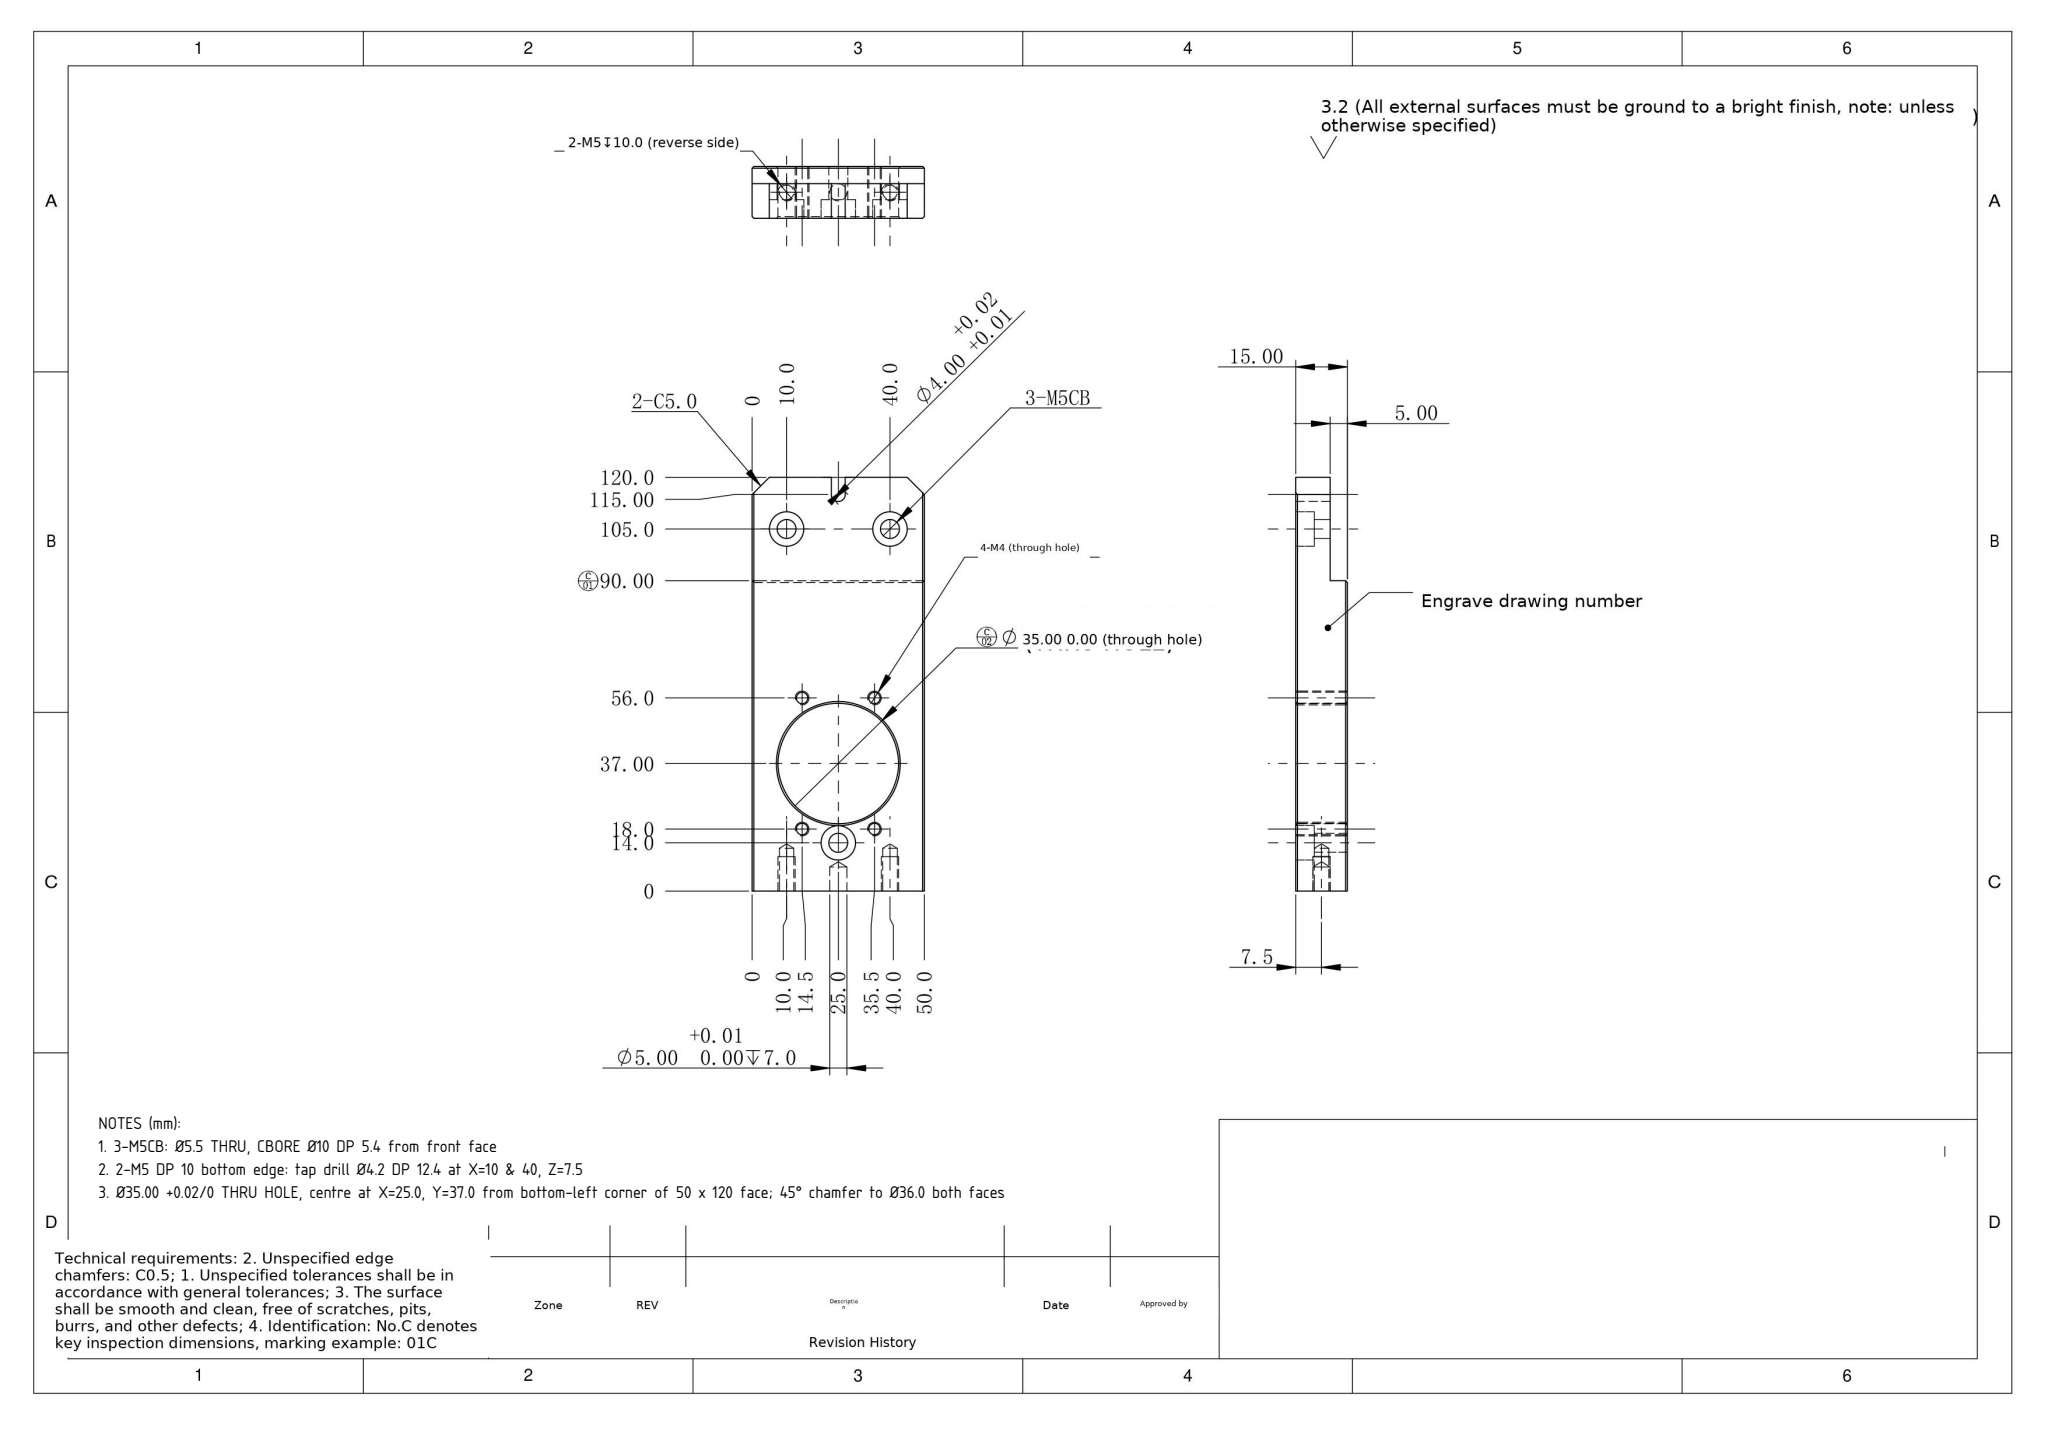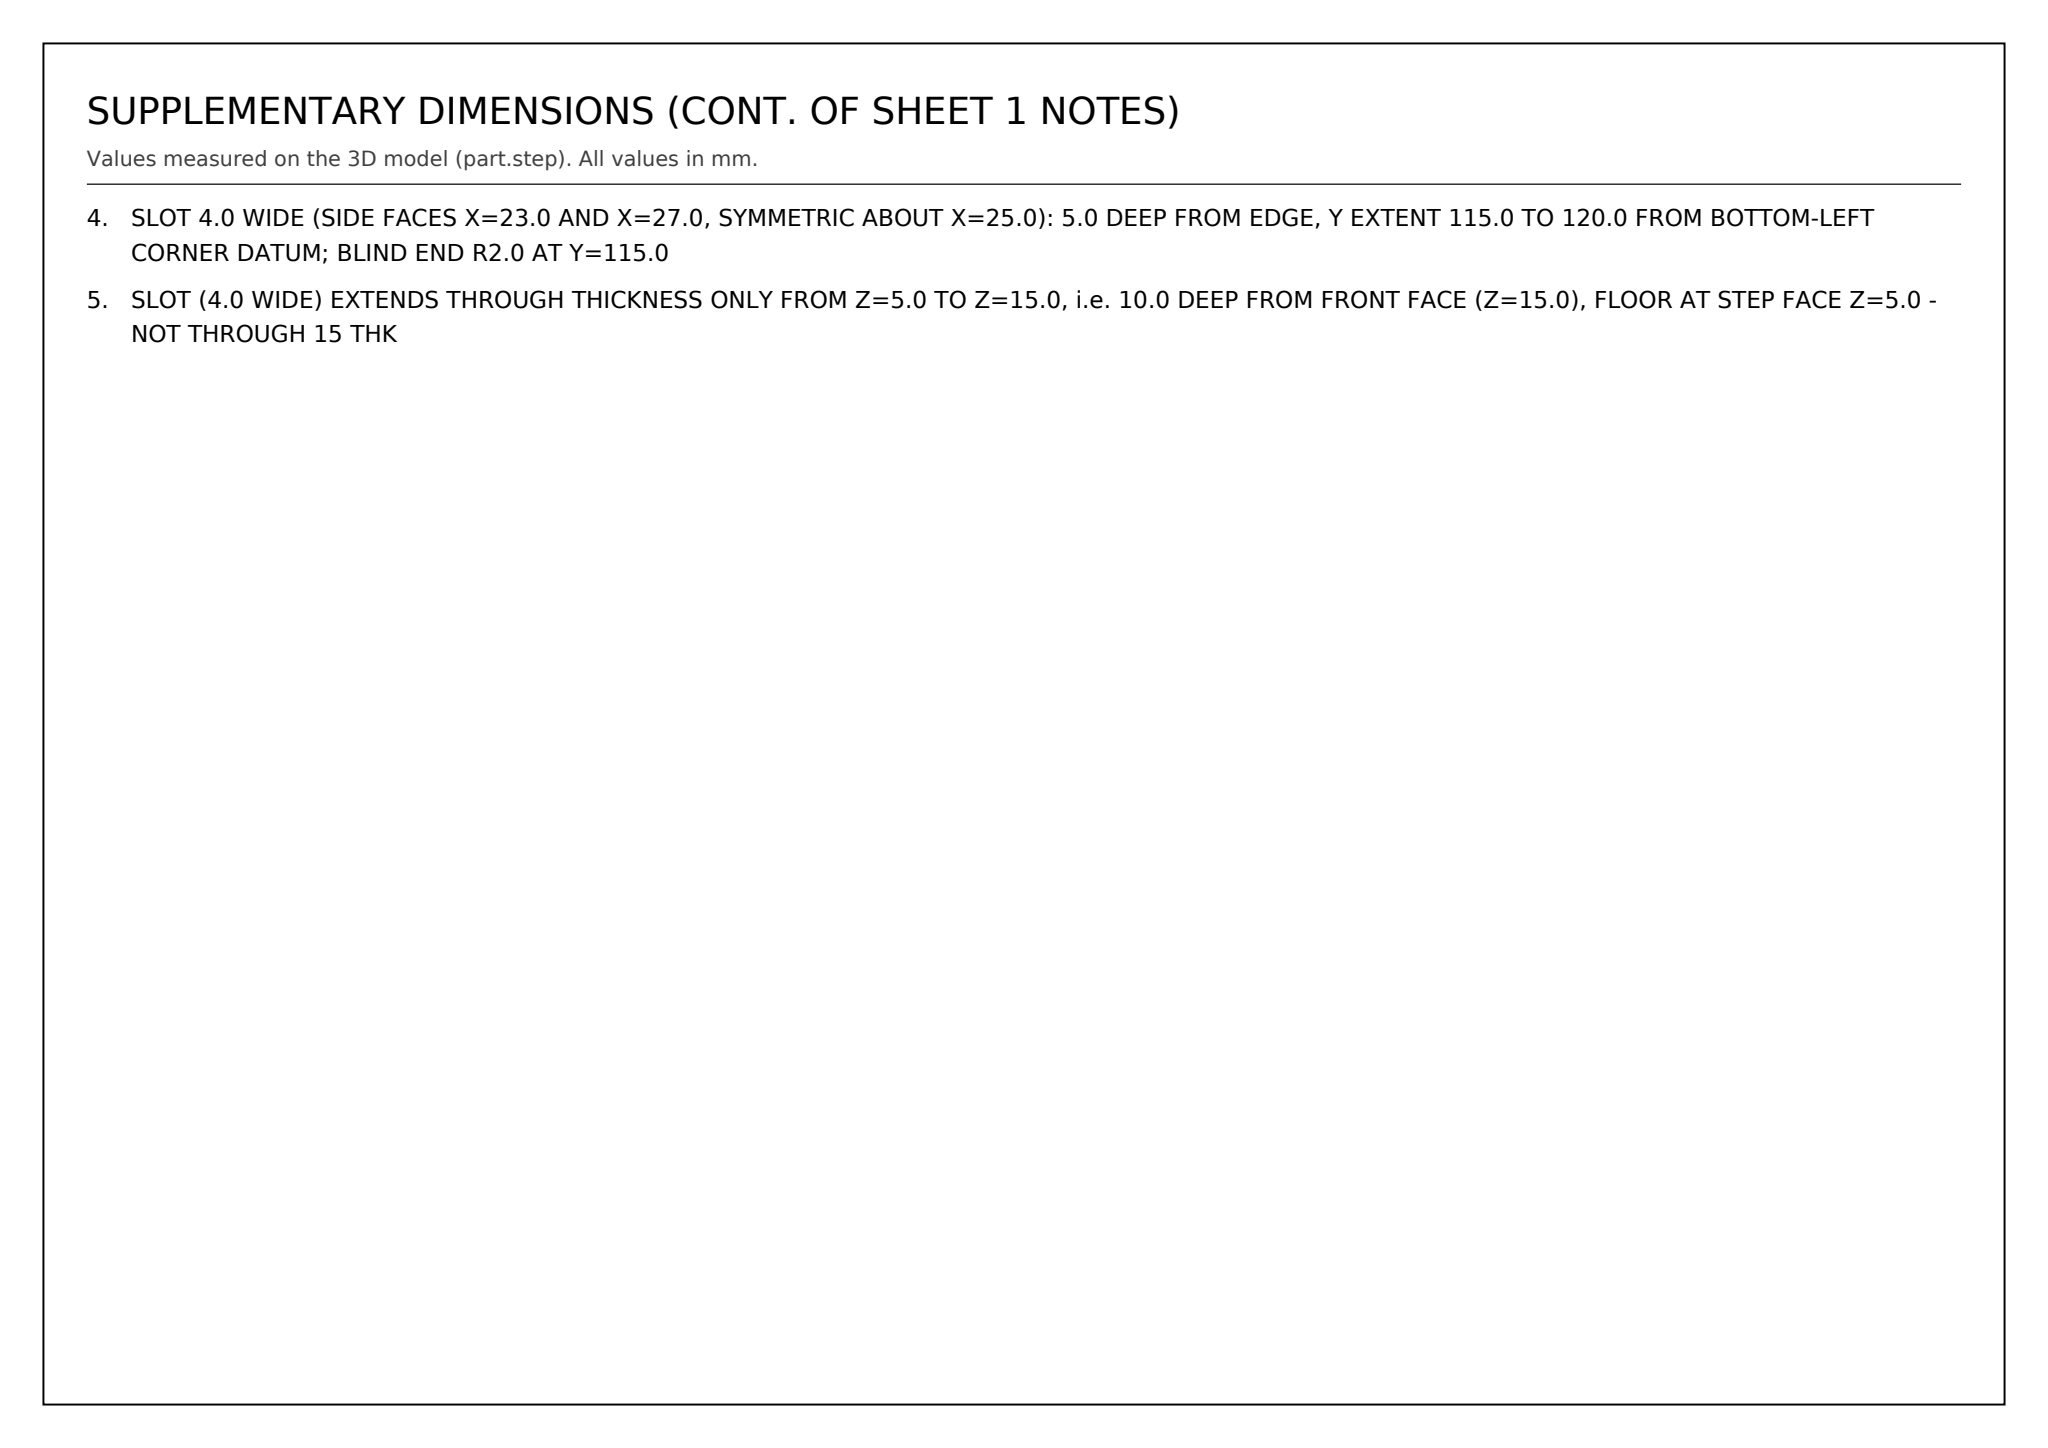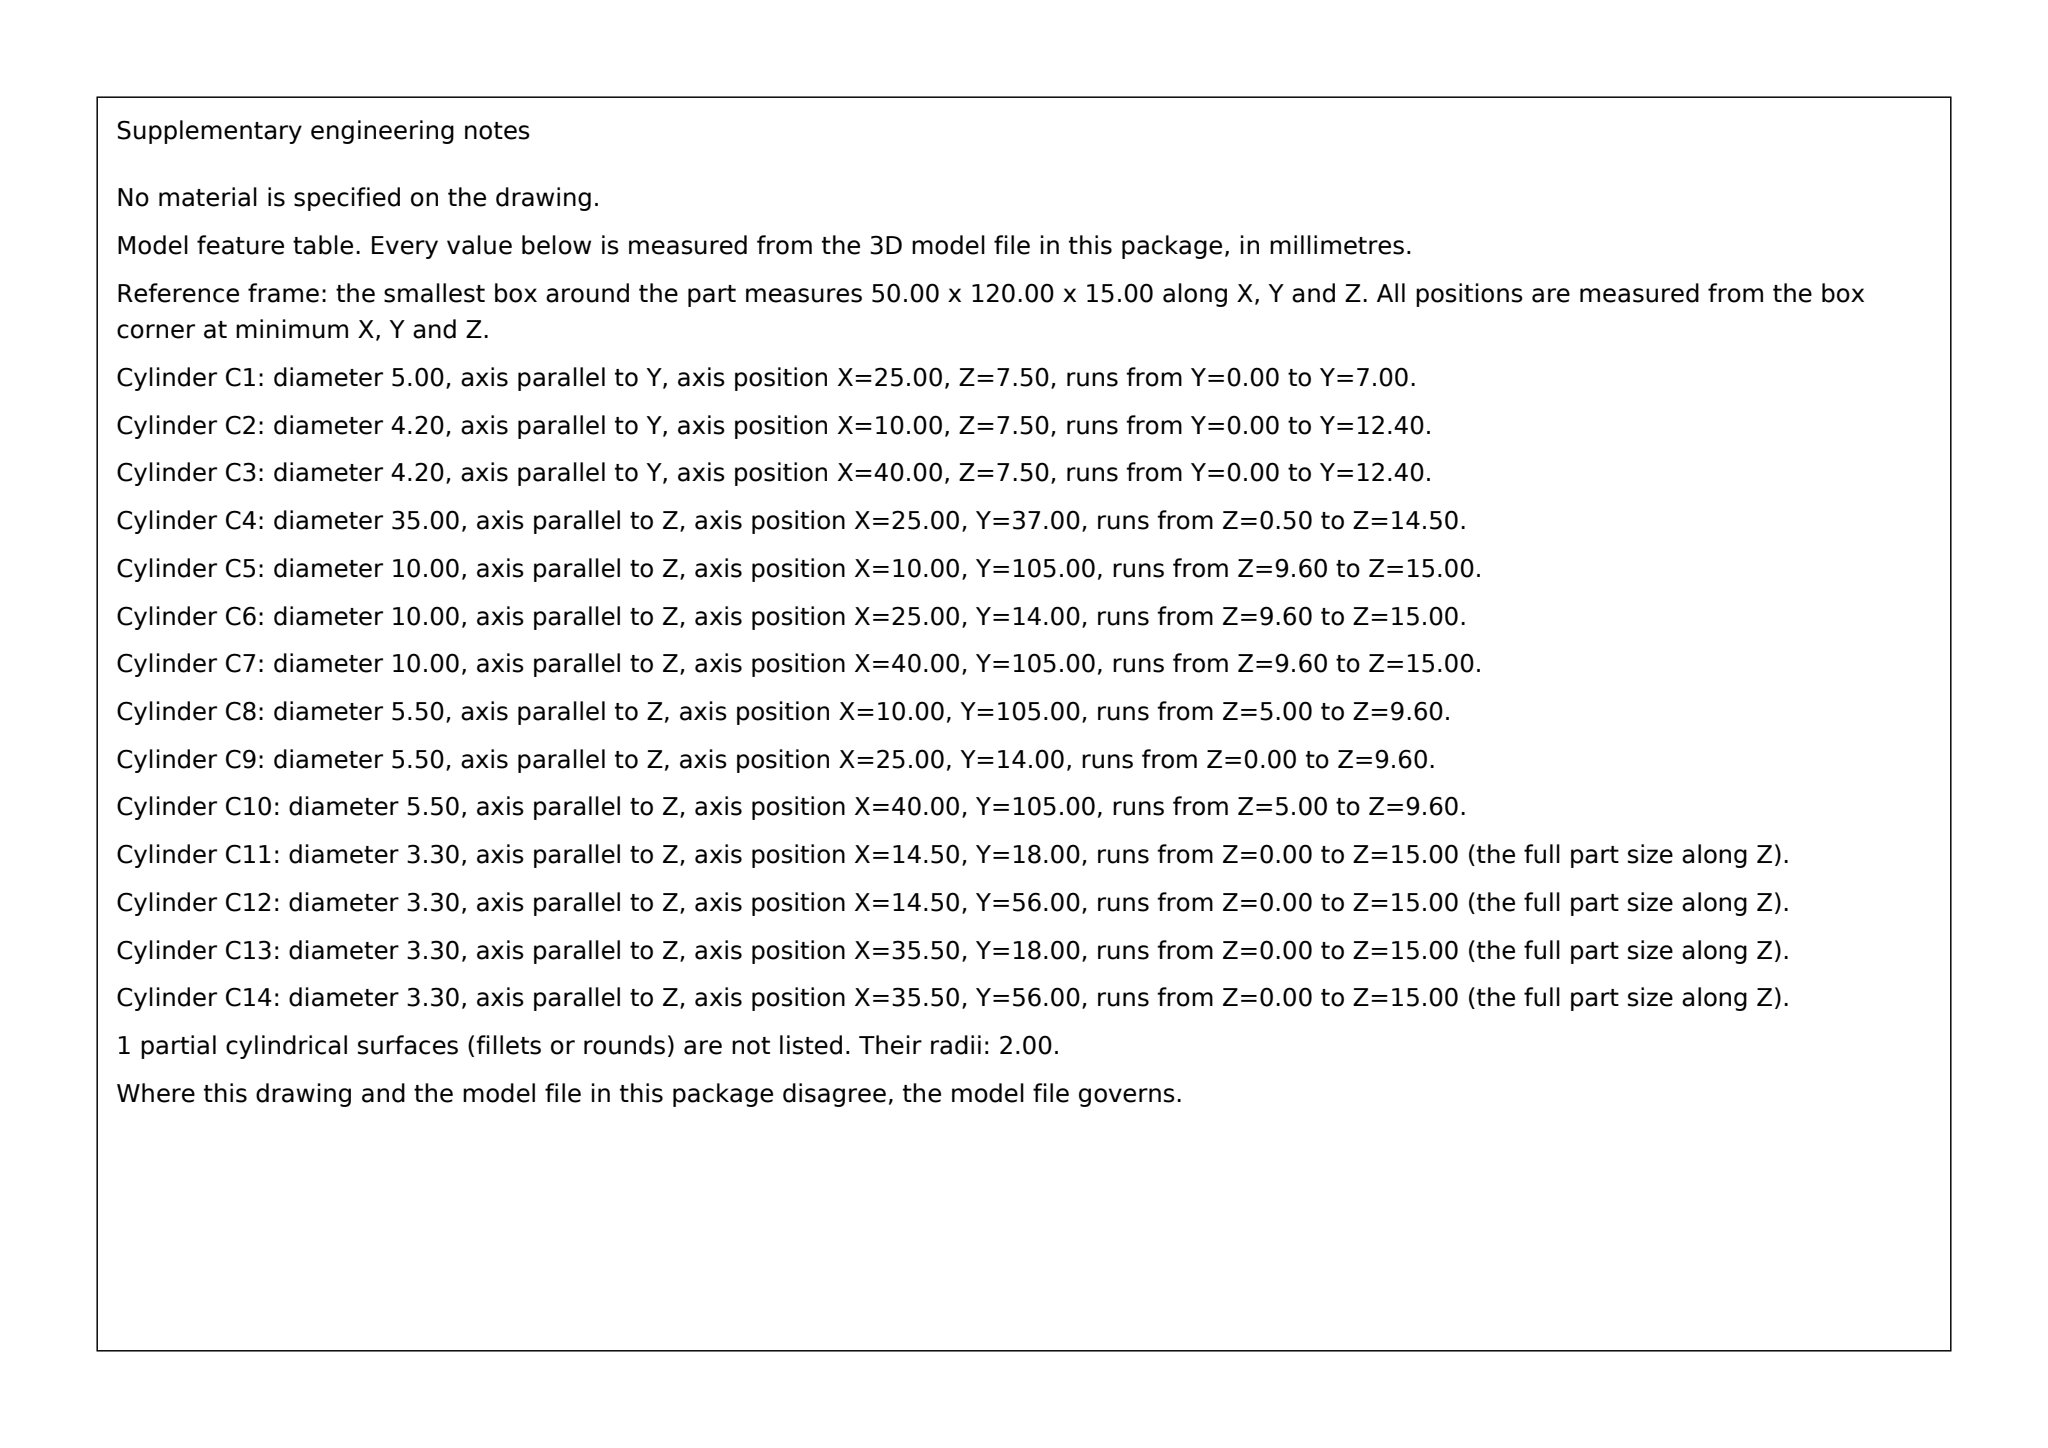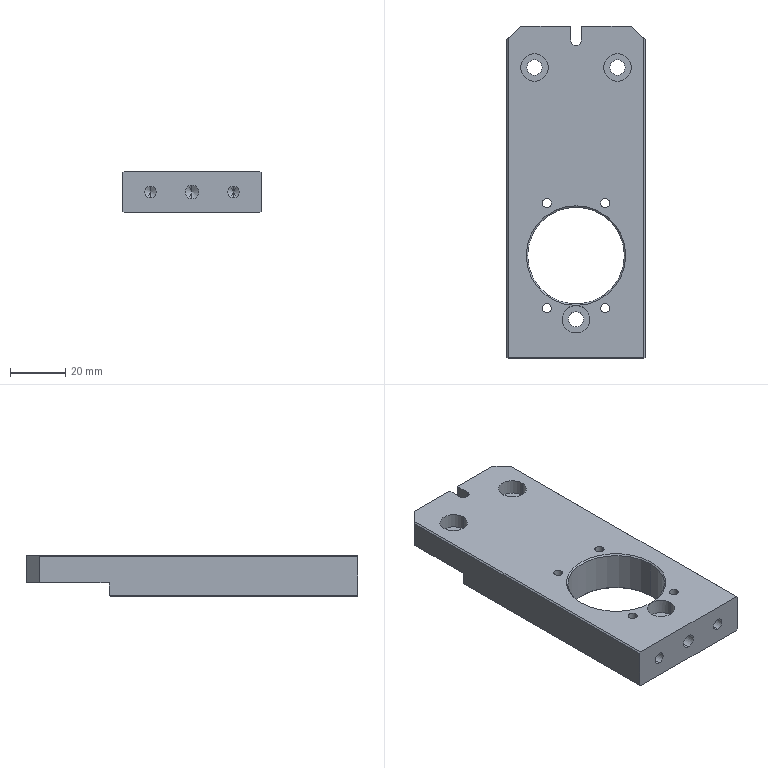Part | SolidWorks | mm | 1 solid | 60 faces | box 50 x 120 x 15 mm | volume 64736 mm3 | cylinder 29 | plane 21 | cone 10 | commonest cylinder face diameters 3.3 x8 10 x6 5.5 x6 4.2 x4 5 x2 35 x2 4 x1
Drawing notes:
3-M5CB: Ø5.5 THRU, CBORE Ø10 DP 5.4 from front face | from the solid: cyl Ø5.5 z L4.6 & Ø10 z L5.4 at (10,105),(40,105); Ø5.5 z L9.6 & Ø10 z L5.4 at (25,14)
2-M5 DP 10 bottom edge: tap drill Ø4.2 DP 12.4 at X=10 & 40, Z=7.5 | from the solid: cyl Ø4.2 axis y at (10,-,7.5) & (40,-,7.5) L12.4; cone 118° ref dia 4.2
Ø35.00 +0.02/0 THRU HOLE, centre at X=25.0, Y=37.0 from bottom-left corner of 50 x 120 face; 45° chamfer to Ø36.0 both faces | from the solid: cylinders: [35.0,"z",[25.0,37.0],14.0]; cones [90.0,35.0] and [90.0,36.0]
SLOT 4.0 WIDE (SIDE FACES X=23.0 AND X=27.0, SYMMETRIC ABOUT X=25.0): 5.0 DEEP FROM EDGE, Y EXTENT 115.0 TO 120.0 FROM BOTTOM-LEFT CORNER DATUM; BLIND END R2.0 AT Y=115.0 | from the solid: axis_planes x=23.0 and x=27.0, extent y [115.0,120.0]; concave arc dia 4.0 axis z at (25.0,115.0)
SLOT (4.0 WIDE) EXTENDS THROUGH THICKNESS ONLY FROM Z=5.0 TO Z=15.0, i.e. 10.0 DEEP FROM FRONT FACE (Z=15.0), FLOOR AT STEP FACE Z=5.0 - NOT THROUGH 15 THK | from the solid: axis_planes x=23.0 / x=27.0 extent z [5.0,15.0]; concave arc dia 4.0 from z=5.0 to z=15.0; plane z=5.0 extent y [90.0,120.0]